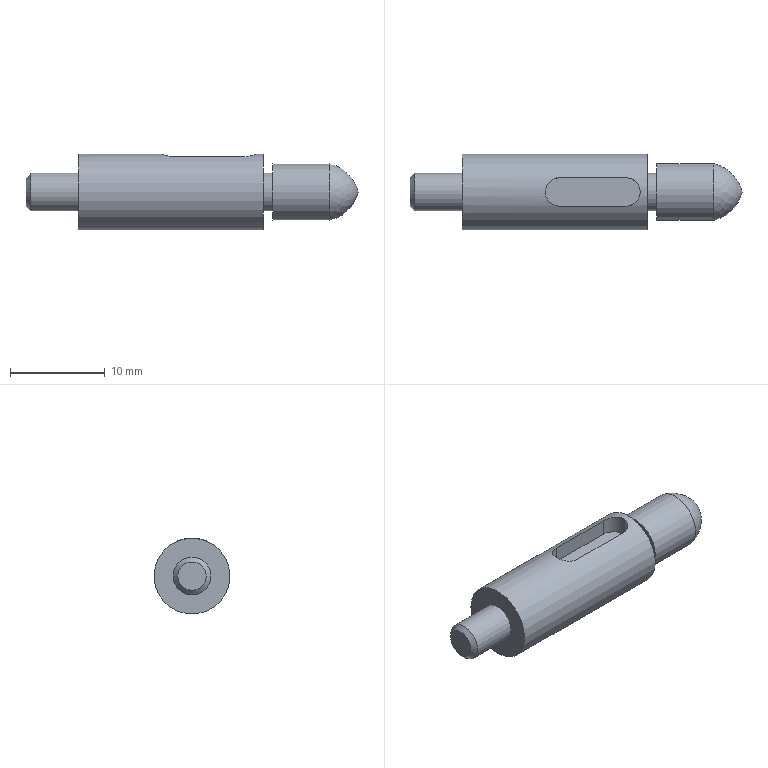Component | NX | ASSY_PRAC_PART_1 | 1 solid | 15 faces | volume 1223 mm3 | plane 7 | cylinder 6 | spline 1 | cone 1 | commonest cylinder face diameters 4 x2 3 x2 6 x1 8 x1